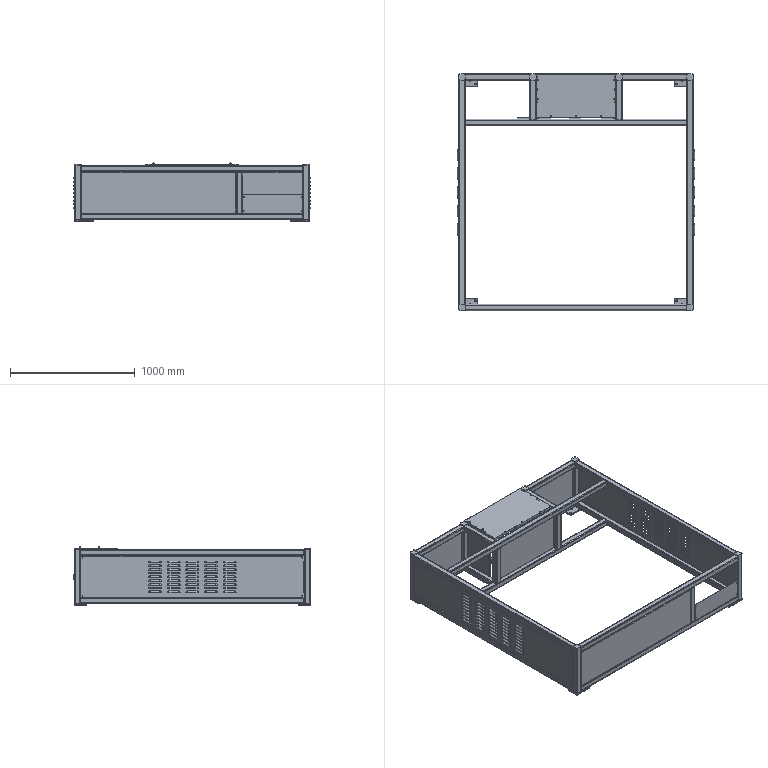Assembly | SolidWorks | mm | 51 component files | 55 solids | 2416 faces | box 1904 x 1905 x 472 mm | volume 47815882 mm3 | plane 1028 | cylinder 680 | sphere 392 | torus 188 | cone 128 | commonest cylinder face diameters 16 x120 6 x100 24 x90 4 x90 28 x90 8 x48 6.8 x32 4.5 x32
Bill of materials:
07.1.1 | 4 |  | Solid rectangular block, elongated, with all four long edges chamfered, giving an octagon-like end cross-section.
19.1.1 | 2 |  | Long, thin sheet-like panel with bent flanges on both long edges (C-shaped profile). It has a central field of raised louvers in five columns of about nine slots each, and small holes near the corners.
20.1.1 | 1 |  | Flat, thin rectangular plate with four oblong slots, two near each short end. It has no other visible features.
21.1.1 | 1 |  | Thin rectangular plate with slightly rounded edges and corners. A small, low raised pad or tab sits on one face, offset toward one edge.
22.1.1 | 1 |  | Thin rectangular plate with slightly rounded edges and corners. A small, low raised pad or tab sits on one face, offset toward one edge (the opposite end from the similar part).
23.1.1 | 1 |  | Plain thin rectangular plate with slightly rounded edges and corners. No holes or protrusions are visible.
24.1.1 | 2 |  | Rectangular sheet-like panel with partial-length folded flanges on all four edges, notched corners, and four small holes near the corners.
25.1.1 | 1 |  | Thin, flat rectangular strip with slightly rounded edges. No other features are visible.
09.1.1 | 4 |  | Long bar with a rectangular cross-section and chamfered longitudinal edges. One end is cut on an angle, tapering the bar's thickness at that end.
AX50x50-1_square tube.1.1 | 6 | AISI 1035 Steel (SS) | Straight prismatic bar with a square cross-section and large-radius rounded corners. It is moderately long compared to its width.
AX50x50-2_square tube.1.1 | 4 | AISI 1035 Steel (SS) | Long, slender, straight bar with a square cross-section and rounded corners. It has flat ends.
AX50x50-3_square tube.1.1 | 4 | AISI 1035 Steel (SS) | Long, slender, straight bar with a rounded-square cross-section and flat ends. Its shape looks very similar to unnamed part.
AX50x50-4_square tube.1.1 | 2 | AISI 1035 Steel (SS) | Long straight solid bar with a square cross-section and rounded longitudinal edges; flat square ends.
AX50x50-5_square tube.1.1 | 3 | AISI 1035 Steel (SS) | Straight solid bar with a square cross-section and rounded longitudinal edges, shown standing upright; flat ends.
AX50x50-6_square tube.1.1 | 4 | AISI 1035 Steel (SS) | Short straight solid bar with a square cross-section and rounded longitudinal edges; flat ends.
AX50x50-8_square tube.1.1 | 2 | AISI 1035 Steel (SS) | Long straight solid bar with a square cross-section and rounded longitudinal edges; flat square ends.
AXWHELL-PLATE.1.1 | 4 |  | Flat rectangular plate with rounded corners. It has four small round through-holes in a 2x2 rectangular pattern and one larger round through-hole near one corner.
04.1.1 | 1 |  | Large thin rectangular plate with slightly rounded corners. Four short tapered pins stick up from one face near the two short edges, and small through-holes run along the edges.
05.1.1 | 4 |  | Long thin flat rectangular strip with a constant thickness. One end is tapered at an angle in plan view, and the cross-section has small chamfered corners.
Mates:
1. coincident | assembly face at (1168.631, -386.636, 222.5) dir (0, 0, -1) | AX00-102.1.1-1/AX00-101.1.1-1/04.1.1-1 face at (-91.369, 1163.364, 222.5) dir (0, 0, 1)
2. coincident | assembly face at (-711.369, 1513.364, 222.5) dir (0, 1, 0) | AX00-102.1.1-1/AX00-101.1.1-1/04.1.1-1 face at (548.631, 1513.364, 222.5) dir (0, 1, 0)
3. coincident | assembly face at (1168.631, -386.636, 242.5) dir (0, 0, 1) | assembly face at (568.631, 1498.364, 242.5) dir (0, 0, -1)
4. coincident | assembly face at (-711.369, 1513.364, 222.5) dir (0, 1, 0) | assembly face at (568.631, 1513.364, 245.5) dir (0, 1, 0)
5. coincident | AX00-100.1.1-1/AXFrame_A.1.1-1/AX50x50-3_square tube.1.1-3 face at (1168.631, 1463.364, 212.5) dir (1, 0, 0) | assembly face at (1168.631, 1498.364, 242.5) dir (1, 0, 0)
6. coincident | AX00-100.1.1-1/AXFrame_A.1.1-1/AX50x50-2_square tube.1.1-5 face at (1118.631, 1148.364, 212.5) dir (0, 1, 0) | 07.1.1-2 face at (-241.369, 1148.364, 158.477) dir (0, -1, 0)
7. coincident | 07.1.1-1 face at (168.631, 1163.364, 188.477) dir (0, 1, 0) | 07.1.1-2 face at (-241.369, 1163.364, 158.477) dir (0, 1, 0)
8. coincident | 07.1.1-1 face at (268.631, 1163.364, 188.477) dir (0, 0, 1) | 07.1.1-2 face at (-141.369, 1148.364, 188.477) dir (0, 0, 1)
9. coincident | assembly face at (1168.631, -386.636, 242.5) dir (0, 0, 1) | assembly face at (261.596, 473.364, 242.5) dir (0, 0, -1)
10. coincident | assembly face at (531.631, 1473.364, 242.5) dir (0, -1, 0) | assembly face at (261.596, 473.364, 642.5) dir (0, 1, 0)
11. coincident | AXFrame_A.1.1-1/AX50x50-1_square tube.1.1-4 face at (1325.438, -406.343, 222.5) dir (1, 0, 0) | 19.1.1-1 face at (1325.438, -353.343, -171.5) dir (1, 0, 0)
12. distance | 19.1.1-1 face at (1323.438, -355.343, 119.5) dir (0, -1, 0) | AXFrame_A.1.1-1/AX50x50-1_square tube.1.1-4 face at (1275.438, -356.343, 222.5) dir (0, 1, 0)
13. distance | 19.1.1-1 face at (1323.438, 1398.657, 161.5) dir (0, 0, 1) | AXFrame_A.1.1-1/AX50x50-3_square tube.1.1-3 face at (1275.438, 1443.657, 162.5) dir (0, 0, -1)
14. coincident | AXFrame_A.1.1-1/AX50x50-1_square tube.1.1-3 face at (-554.562, -406.343, 222.5) dir (-1, 0, 0) | 19.1.1-2 face at (-554.562, 1440.657, -171.5) dir (-1, 0, 0)
15. distance | 19.1.1-2 face at (-552.562, -311.343, 161.5) dir (0, 0, 1) | AXFrame_A.1.1-1/AX50x50-3_square tube.1.1-1 face at (-554.562, 1443.657, 162.5) dir (0, 0, -1)
16. distance | 19.1.1-2 face at (-552.562, 1442.657, 119.5) dir (0, 1, 0) | AXFrame_A.1.1-1/AX50x50-1_square tube.1.1-6 face at (-554.562, 1443.657, 222.5) dir (0, -1, 0)
17. coincident | AXFrame_A.1.1-1/AX50x50-8_square tube.1.1-3 face at (755.438, 1493.657, -222.5) dir (0, 1, 0) | 21.1.1-1 face at (756.438, 1493.657, 161.5) dir (0, 1, 0)
18. distance | 21.1.1-1 face at (1274.438, 1493.657, 161.5) dir (0, 0, 1) | AXFrame_A.1.1-1/AX50x50-8_square tube.1.1-4 face at (755.438, 1443.657, 162.5) dir (0, 0, -1)
19. distance | 21.1.1-1 face at (756.438, 1493.657, -171.5) dir (-1, 0, 0) | AXFrame_A.1.1-1/AX50x50-1_square tube.1.1-7 face at (755.438, 1443.657, 222.5) dir (1, 0, 0)
20. coincident | AXFrame_A.1.1-1/AX50x50-4_square tube.1.1-3 face at (-504.562, 1493.657, -222.5) dir (0, 1, 0) | 22.1.1-2 face at (14.438, 1493.657, -171.5) dir (0, 1, 0)
21. distance | 22.1.1-2 face at (-503.562, 1493.657, 161.5) dir (-1, 0, 0) | AXFrame_A.1.1-1/AX50x50-1_square tube.1.1-6 face at (-504.562, 1443.657, 222.5) dir (1, 0, 0)
22. distance | 22.1.1-2 face at (-503.562, 1493.657, 161.5) dir (0, 0, 1) | AXFrame_A.1.1-1/AX50x50-4_square tube.1.1-4 face at (-504.562, 1443.657, 162.5) dir (0, 0, -1)
23. coincident | AXFrame_A.1.1-1/AX50x50-5_square tube.1.1-1 face at (15.438, 1128.657, 162.5) dir (0, 1, 0) | 23.1.1-1 face at (704.438, 1128.657, -170.5) dir (0, 1, 0)
24. coincident | AXFrame_A.1.1-1/AX50x50-2_square tube.1.1-5 face at (1275.438, 1078.657, 162.5) dir (0, 0, -1) | 23.1.1-1 face at (66.438, 1128.657, 162.5) dir (0, 0, 1)
25. distance | 23.1.1-1 face at (704.438, 1128.657, 162.5) dir (1, 0, 0) | AXFrame_A.1.1-1/AX50x50-5_square tube.1.1-2 face at (705.438, 1078.657, 162.5) dir (-1, 0, 0)
26. coincident | AXFrame_A.1.1-1/AX50x50-1_square tube.1.1-7 face at (705.438, 1443.657, 222.5) dir (-1, 0, 0) | 24.1.1-1 face at (705.438, 1374.657, -171.5) dir (-1, 0, 0)
27. distance | AXFrame_A.1.1-1/AX50x50-5_square tube.1.1-2 face at (705.438, 1128.657, 162.5) dir (0, 1, 0) | 24.1.1-1 face at (707.438, 1129.657, -129.5) dir (0, -1, 0)
28. distance | 24.1.1-1 face at (707.438, 1332.657, -171.5) dir (0, 0, -1) | AXFrame_A.1.1-1/AX50x50-6_square tube.1.1-4 face at (705.438, 1128.657, -172.5) dir (0, 0, 1)
29. coincident | AXFrame_A.1.1-1/AX50x50-1_square tube.1.1-8 face at (65.438, 1443.657, 222.5) dir (1, 0, 0) | 24.1.1-2 face at (65.438, 1197.657, -171.5) dir (1, 0, 0)
30. distance | 24.1.1-2 face at (63.438, 1398.657, 161.5) dir (0, 0, 1) | AXFrame_A.1.1-1/AX50x50-6_square tube.1.1-1 face at (15.438, 1128.657, 162.5) dir (0, 0, -1)
31. distance | 24.1.1-2 face at (63.438, 1442.657, -129.5) dir (0, 1, 0) | AXFrame_A.1.1-1/AX50x50-1_square tube.1.1-8 face at (15.438, 1443.657, 222.5) dir (0, -1, 0)
32. coincident | AXFrame_A.1.1-1/AX50x50-2_square tube.1.1-3 face at (1275.438, -406.343, -172.5) dir (0, -1, 0) | 25.1.1-1 face at (739.438, -406.343, 161.5) dir (0, -1, 0)
33. distance | 25.1.1-1 face at (-503.562, -406.343, -171.5) dir (-1, 0, 0) | AXFrame_A.1.1-1/AX50x50-1_square tube.1.1-3 face at (-504.562, -406.343, 222.5) dir (1, 0, 0)
34. distance | 25.1.1-1 face at (-503.562, -406.343, 161.5) dir (0, 0, 1) | AXFrame_A.1.1-1/AX50x50-2_square tube.1.1-2 face at (1275.438, -406.343, 162.5) dir (0, 0, -1)
35. coincident | AX50x50-1_square tube.1.1-3 face at (22.742, -23.319, 222.5) dir (1, 0, 0) | AX50x50-2_square tube.1.1-2 face at (22.742, 26.681, 162.5) dir (-1, 0, 0)
36. coincident | AX50x50-1_square tube.1.1-3 face at (-27.258, -23.319, 222.5) dir (0, -1, 0) | AX50x50-2_square tube.1.1-2 face at (1802.742, -23.319, 212.5) dir (0, -1, 0)
37. distance | AX50x50-1_square tube.1.1-3 face at (22.742, 26.681, 222.5) dir (0, 0, 1) | AX50x50-2_square tube.1.1-2 face at (1802.742, -23.319, 212.5) dir (0, 0, 1)
38. coincident | AX50x50-2_square tube.1.1-2 face at (1802.742, 26.681, 162.5) dir (1, 0, 0) | AX50x50-1_square tube.1.1-4 face at (1802.742, -23.319, 222.5) dir (-1, 0, 0)
39. coincident | AX50x50-2_square tube.1.1-2 face at (1802.742, -23.319, 212.5) dir (0, -1, 0) | AX50x50-1_square tube.1.1-4 face at (1802.742, -23.319, 222.5) dir (0, -1, 0)
40. coincident | AX50x50-1_square tube.1.1-3 face at (22.742, -23.319, 222.5) dir (1, 0, 0) | AX50x50-2_square tube.1.1-3 face at (22.742, 26.681, -222.5) dir (-1, 0, 0)
41. coincident | AX50x50-1_square tube.1.1-3 face at (-27.258, -23.319, 222.5) dir (0, -1, 0) | AX50x50-2_square tube.1.1-3 face at (1802.742, -23.319, -172.5) dir (0, -1, 0)
42. coincident | AX50x50-1_square tube.1.1-3 face at (22.742, 26.681, -222.5) dir (0, 0, -1) | AX50x50-2_square tube.1.1-3 face at (1802.742, -23.319, -222.5) dir (0, 0, -1)
43. coincident | AX50x50-1_square tube.1.1-3 face at (-27.258, 26.681, 222.5) dir (0, 1, 0) | AX50x50-3_square tube.1.1-1 face at (22.742, 26.681, 162.5) dir (0, -1, 0)
44. coincident | AX50x50-1_square tube.1.1-3 face at (-27.258, -23.319, 222.5) dir (-1, 0, 0) | AX50x50-3_square tube.1.1-1 face at (-27.258, 1826.681, 212.5) dir (-1, 0, 0)
45. distance | AX50x50-1_square tube.1.1-3 face at (22.742, 26.681, 222.5) dir (0, 0, 1) | AX50x50-3_square tube.1.1-1 face at (-27.258, 1826.681, 212.5) dir (0, 0, 1)
46. coincident | AX50x50-1_square tube.1.1-3 face at (-27.258, 26.681, 222.5) dir (0, 1, 0) | AX50x50-3_square tube.1.1-2 face at (22.742, 26.681, -222.5) dir (0, -1, 0)
47. coincident | AX50x50-1_square tube.1.1-3 face at (22.742, 26.681, -222.5) dir (0, 0, -1) | AX50x50-3_square tube.1.1-2 face at (-27.258, 1826.681, -222.5) dir (0, 0, -1)
48. coincident | AX50x50-1_square tube.1.1-3 face at (-27.258, -23.319, 222.5) dir (-1, 0, 0) | AX50x50-3_square tube.1.1-2 face at (-27.258, 1826.681, -172.5) dir (-1, 0, 0)
49. coincident | AX50x50-1_square tube.1.1-4 face at (1802.742, 26.681, 222.5) dir (0, 1, 0) | AX50x50-3_square tube.1.1-3 face at (1852.742, 26.681, 162.5) dir (0, -1, 0)
50. distance | AX50x50-1_square tube.1.1-4 face at (1852.742, 26.681, 222.5) dir (0, 0, 1) | AX50x50-3_square tube.1.1-3 face at (1802.742, 1826.681, 212.5) dir (0, 0, 1)
51. coincident | AX50x50-1_square tube.1.1-4 face at (1852.742, -23.319, 222.5) dir (1, 0, 0) | AX50x50-3_square tube.1.1-3 face at (1852.742, 1826.681, 212.5) dir (1, 0, 0)
52. coincident | AX50x50-1_square tube.1.1-4 face at (1852.742, -23.319, 222.5) dir (1, 0, 0) | AX50x50-3_square tube.1.1-4 face at (1852.742, 1826.681, -172.5) dir (1, 0, 0)
53. coincident | AX50x50-1_square tube.1.1-4 face at (1802.742, 26.681, 222.5) dir (0, 1, 0) | AX50x50-3_square tube.1.1-4 face at (1852.742, 26.681, -222.5) dir (0, -1, 0)
54. coincident | AX50x50-1_square tube.1.1-4 face at (1852.742, 26.681, -222.5) dir (0, 0, -1) | AX50x50-3_square tube.1.1-4 face at (1802.742, 1826.681, -222.5) dir (0, 0, -1)
55. coincident | AX50x50-1_square tube.1.1-3 face at (22.742, 26.681, -222.5) dir (0, 0, -1) | AX50x50-1_square tube.1.1-4 face at (1852.742, 26.681, -222.5) dir (0, 0, -1)
56. coincident | AX50x50-1_square tube.1.1-4 face at (1852.742, 26.681, 222.5) dir (0, 0, 1) | AX50x50-1_square tube.1.1-5 face at (1852.742, 1876.681, 222.5) dir (0, 0, 1)
57. coincident | AX50x50-3_square tube.1.1-3 face at (1852.742, 1826.681, 212.5) dir (1, 0, 0) | AX50x50-1_square tube.1.1-5 face at (1852.742, 1826.681, 222.5) dir (1, 0, 0)
58. coincident | AX50x50-3_square tube.1.1-3 face at (1852.742, 1826.681, 162.5) dir (0, 1, 0) | AX50x50-1_square tube.1.1-5 edge at (1810.742, 1826.681, 222.5) dir (0, 0, -1)
59. coincident | AX50x50-3_square tube.1.1-1 face at (22.742, 1826.681, 212.5) dir (1, 0, 0) | AX50x50-1_square tube.1.1-6 face at (22.742, 1826.681, 222.5) dir (1, 0, 0)
60. coincident | AX50x50-1_square tube.1.1-3 face at (22.742, 26.681, 222.5) dir (0, 0, 1) | AX50x50-1_square tube.1.1-6 face at (22.742, 1876.681, 222.5) dir (0, 0, 1)
61. coincident | AX50x50-3_square tube.1.1-1 face at (22.742, 1826.681, 162.5) dir (0, 1, 0) | AX50x50-1_square tube.1.1-6 face at (-27.258, 1826.681, 222.5) dir (0, -1, 0)
62. coincident | AX50x50-3_square tube.1.1-4 face at (1802.742, 1826.681, -172.5) dir (-1, 0, 0) | AX50x50-2_square tube.1.1-4 face at (1802.742, 1511.681, -222.5) dir (1, 0, 0)
63. coincident | AX50x50-3_square tube.1.1-4 face at (1802.742, 1826.681, -222.5) dir (0, 0, -1) | AX50x50-2_square tube.1.1-4 face at (1802.742, 1461.681, -222.5) dir (0, 0, -1)
64. coincident | AX50x50-3_square tube.1.1-3 face at (1802.742, 1826.681, 212.5) dir (-1, 0, 0) | AX50x50-2_square tube.1.1-5 face at (1802.742, 1511.681, 162.5) dir (1, 0, 0)
65. coincident | AX50x50-3_square tube.1.1-3 face at (1802.742, 1826.681, 212.5) dir (0, 0, 1) | AX50x50-2_square tube.1.1-5 face at (1802.742, 1461.681, 212.5) dir (0, 0, 1)
66. coincident | AX50x50-2_square tube.1.1-4 face at (1802.742, 1511.681, -172.5) dir (0, 1, 0) | AX50x50-2_square tube.1.1-5 face at (1802.742, 1511.681, 212.5) dir (0, 1, 0)
67. coincident | AX50x50-1_square tube.1.1-5 face at (1802.742, 1826.681, 222.5) dir (-1, 0, 0) | AX50x50-8_square tube.1.1-3 face at (1802.742, 1876.681, -172.5) dir (1, 0, 0)
68. coincident | AX50x50-1_square tube.1.1-5 face at (1802.742, 1876.681, 222.5) dir (0, 1, 0) | AX50x50-8_square tube.1.1-3 face at (1282.742, 1876.681, -222.5) dir (0, 1, 0)
69. coincident | AX50x50-1_square tube.1.1-5 face at (1852.742, 1876.681, -222.5) dir (0, 0, -1) | AX50x50-8_square tube.1.1-3 face at (1282.742, 1826.681, -222.5) dir (0, 0, -1)
70. coincident | AX50x50-1_square tube.1.1-5 face at (1802.742, 1876.681, 222.5) dir (0, 1, 0) | AX50x50-8_square tube.1.1-4 face at (1282.742, 1876.681, 162.5) dir (0, 1, 0)
71. coincident | AX50x50-1_square tube.1.1-5 face at (1802.742, 1826.681, 222.5) dir (-1, 0, 0) | AX50x50-8_square tube.1.1-4 face at (1802.742, 1876.681, 212.5) dir (1, 0, 0)
72. coincident | AX50x50-1_square tube.1.1-6 face at (-27.258, 1876.681, 222.5) dir (0, 1, 0) | AX50x50-4_square tube.1.1-3 face at (22.742, 1876.681, -222.5) dir (0, 1, 0)
73. coincident | AX50x50-1_square tube.1.1-6 face at (22.742, 1876.681, -222.5) dir (0, 0, -1) | AX50x50-4_square tube.1.1-3 face at (22.742, 1826.681, -222.5) dir (0, 0, -1)
74. coincident | AX50x50-1_square tube.1.1-6 face at (22.742, 1826.681, 222.5) dir (1, 0, 0) | AX50x50-4_square tube.1.1-3 face at (22.742, 1876.681, -172.5) dir (-1, 0, 0)
75. coincident | AX50x50-1_square tube.1.1-6 face at (22.742, 1826.681, 222.5) dir (1, 0, 0) | AX50x50-4_square tube.1.1-4 face at (22.742, 1876.681, 212.5) dir (-1, 0, 0)
76. coincident | AX50x50-1_square tube.1.1-6 face at (-27.258, 1876.681, 222.5) dir (0, 1, 0) | AX50x50-4_square tube.1.1-4 face at (22.742, 1876.681, 162.5) dir (0, 1, 0)
77. coincident | AX50x50-3_square tube.1.1-1 face at (-27.258, 1826.681, 212.5) dir (0, 0, 1) | AX50x50-4_square tube.1.1-4 face at (22.742, 1826.681, 212.5) dir (0, 0, 1)
78. coincident | AX50x50-3_square tube.1.1-3 face at (1802.742, 1826.681, 212.5) dir (0, 0, 1) | AX50x50-8_square tube.1.1-4 face at (1282.742, 1826.681, 212.5) dir (0, 0, 1)
79. coincident | AX50x50-1_square tube.1.1-5 face at (1852.742, 1876.681, 222.5) dir (0, 0, 1) | AX50x50-1_square tube.1.1-7 face at (1282.742, 1876.681, 222.5) dir (0, 0, 1)
80. coincident | AX50x50-8_square tube.1.1-4 face at (1282.742, 1876.681, 162.5) dir (0, 1, 0) | AX50x50-1_square tube.1.1-7 face at (1232.742, 1876.681, 222.5) dir (0, 1, 0)
81. coincident | AX50x50-8_square tube.1.1-4 face at (1282.742, 1876.681, 212.5) dir (-1, 0, 0) | AX50x50-1_square tube.1.1-7 face at (1282.742, 1826.681, 222.5) dir (1, 0, 0)
82. coincident | AX50x50-4_square tube.1.1-4 face at (22.742, 1876.681, 162.5) dir (0, 1, 0) | AX50x50-1_square tube.1.1-8 face at (542.742, 1876.681, 222.5) dir (0, 1, 0)
83. coincident | AX50x50-1_square tube.1.1-7 face at (1282.742, 1876.681, 222.5) dir (0, 0, 1) | AX50x50-1_square tube.1.1-8 face at (592.742, 1876.681, 222.5) dir (0, 0, 1)
84. coincident | AX50x50-4_square tube.1.1-4 face at (542.742, 1876.681, 212.5) dir (1, 0, 0) | AX50x50-1_square tube.1.1-8 face at (542.742, 1826.681, 222.5) dir (-1, 0, 0)
85. coincident | AX50x50-1_square tube.1.1-8 face at (542.742, 1826.681, 222.5) dir (0, -1, 0) | AX50x50-6_square tube.1.1-1 face at (592.742, 1826.681, 212.5) dir (0, 1, 0)
86. coincident | AX50x50-1_square tube.1.1-8 face at (592.742, 1826.681, 222.5) dir (1, 0, 0) | AX50x50-6_square tube.1.1-1 face at (592.742, 1511.681, 162.5) dir (1, 0, 0)
87. coincident | AX50x50-1_square tube.1.1-8 face at (542.742, 1826.681, 222.5) dir (0, -1, 0) | AX50x50-6_square tube.1.1-2 face at (592.742, 1826.681, -222.5) dir (0, 1, 0)
88. coincident | AX50x50-1_square tube.1.1-8 face at (592.742, 1826.681, 222.5) dir (1, 0, 0) | AX50x50-6_square tube.1.1-2 face at (592.742, 1511.681, -172.5) dir (1, 0, 0)
89. coincident | AX50x50-1_square tube.1.1-8 face at (592.742, 1876.681, -222.5) dir (0, 0, -1) | AX50x50-6_square tube.1.1-2 face at (542.742, 1511.681, -222.5) dir (0, 0, -1)
90. coincident | AX50x50-1_square tube.1.1-7 face at (1282.742, 1826.681, 222.5) dir (1, 0, 0) | AX50x50-6_square tube.1.1-3 face at (1282.742, 1511.681, 212.5) dir (1, 0, 0)
91. coincident | AX50x50-1_square tube.1.1-7 face at (1282.742, 1826.681, 222.5) dir (1, 0, 0) | AX50x50-6_square tube.1.1-4 face at (1282.742, 1511.681, -172.5) dir (1, 0, 0)
92. coincident | AX50x50-2_square tube.1.1-5 face at (1802.742, 1461.681, 212.5) dir (0, 0, 1) | AX50x50-6_square tube.1.1-1 face at (542.742, 1511.681, 212.5) dir (0, 0, 1)
93. coincident | AX50x50-1_square tube.1.1-7 face at (1232.742, 1826.681, 222.5) dir (0, -1, 0) | AX50x50-6_square tube.1.1-3 face at (1282.742, 1826.681, 162.5) dir (0, 1, 0)
94. coincident | AX50x50-2_square tube.1.1-5 face at (1802.742, 1461.681, 212.5) dir (0, 0, 1) | AX50x50-6_square tube.1.1-3 face at (1232.742, 1511.681, 212.5) dir (0, 0, 1)
95. coincident | AX50x50-1_square tube.1.1-7 face at (1232.742, 1826.681, 222.5) dir (0, -1, 0) | AX50x50-6_square tube.1.1-4 face at (1282.742, 1826.681, -222.5) dir (0, 1, 0)
96. coincident | AX50x50-1_square tube.1.1-7 face at (1282.742, 1876.681, -222.5) dir (0, 0, -1) | AX50x50-6_square tube.1.1-4 face at (1232.742, 1511.681, -222.5) dir (0, 0, -1)
97. coincident | AX50x50-2_square tube.1.1-4 face at (1802.742, 1511.681, -172.5) dir (0, 1, 0) | AX50x50-6_square tube.1.1-4 face at (1282.742, 1511.681, -222.5) dir (0, -1, 0)
98. coincident | AX50x50-2_square tube.1.1-4 face at (1802.742, 1511.681, -172.5) dir (0, 1, 0) | AX50x50-5_square tube.1.1-1 face at (542.742, 1511.681, 162.5) dir (0, 1, 0)
99. coincident | AX50x50-6_square tube.1.1-2 face at (592.742, 1511.681, -172.5) dir (1, 0, 0) | AX50x50-5_square tube.1.1-1 face at (592.742, 1461.681, 162.5) dir (1, 0, 0)
100. coincident | AX50x50-2_square tube.1.1-4 face at (1802.742, 1461.681, -172.5) dir (0, 0, 1) | AX50x50-5_square tube.1.1-1 face at (592.742, 1511.681, -172.5) dir (0, 0, -1)
101. coincident | AX50x50-2_square tube.1.1-4 face at (1802.742, 1511.681, -172.5) dir (0, 1, 0) | AX50x50-5_square tube.1.1-2 face at (1232.742, 1511.681, 162.5) dir (0, 1, 0)
102. coincident | AX50x50-2_square tube.1.1-4 face at (1802.742, 1461.681, -172.5) dir (0, 0, 1) | AX50x50-5_square tube.1.1-2 face at (1282.742, 1511.681, -172.5) dir (0, 0, -1)
103. coincident | AX50x50-6_square tube.1.1-3 face at (1232.742, 1511.681, 212.5) dir (-1, 0, 0) | AX50x50-5_square tube.1.1-2 face at (1232.742, 1461.681, 162.5) dir (-1, 0, 0)
104. coincident | AX50x50-1_square tube.1.1-4 face at (1852.742, 26.681, -222.5) dir (0, 0, -1) | AXwheel-assembly-2.1.1-2/AXWHELL-PLATE.1.1-1 face at (1852.742, -23.319, -222.5) dir (0, 0, 1)
105. coincident | AX50x50-1_square tube.1.1-4 face at (1802.742, -23.319, 222.5) dir (0, -1, 0) | AXwheel-assembly-2.1.1-2/AXWHELL-PLATE.1.1-1 face at (1702.742, -23.319, -222.5) dir (0, -1, 0)
106. coincident | AX50x50-1_square tube.1.1-4 face at (1852.742, -23.319, 222.5) dir (1, 0, 0) | AXwheel-assembly-2.1.1-2/AXWHELL-PLATE.1.1-1 face at (1852.742, -23.319, -222.5) dir (1, 0, 0)
107. coincident | AX50x50-1_square tube.1.1-3 face at (22.742, 26.681, -222.5) dir (0, 0, -1) | AXwheel-assembly-1.1.1-2/AXWHELL-PLATE.1.1-1 face at (-27.258, -23.319, -222.5) dir (0, 0, 1)
108. coincident | AX50x50-1_square tube.1.1-3 face at (-27.258, -23.319, 222.5) dir (0, -1, 0) | AXwheel-assembly-1.1.1-2/AXWHELL-PLATE.1.1-1 face at (122.742, -23.319, -234.5) dir (0, -1, 0)
109. coincident | AX50x50-1_square tube.1.1-3 face at (-27.258, -23.319, 222.5) dir (-1, 0, 0) | AXwheel-assembly-1.1.1-2/AXWHELL-PLATE.1.1-1 face at (-27.258, -23.319, -234.5) dir (-1, 0, 0)
110. coincident | AX50x50-1_square tube.1.1-6 face at (22.742, 1876.681, -222.5) dir (0, 0, -1) | AXwheel-assembly-3.1.1-2/AXWHELL-PLATE.1.1-1 face at (-27.258, 1876.681, -222.5) dir (0, 0, 1)
111. coincident | AX50x50-1_square tube.1.1-6 face at (-27.258, 1826.681, 222.5) dir (-1, 0, 0) | AXwheel-assembly-3.1.1-2/AXWHELL-PLATE.1.1-1 face at (-27.258, 1876.681, -222.5) dir (-1, 0, 0)
112. coincident | AX50x50-1_square tube.1.1-6 face at (-27.258, 1876.681, 222.5) dir (0, 1, 0) | AXwheel-assembly-3.1.1-2/AXWHELL-PLATE.1.1-1 face at (122.742, 1876.681, -222.5) dir (0, 1, 0)
113. coincident | AX50x50-1_square tube.1.1-5 face at (1852.742, 1876.681, -222.5) dir (0, 0, -1) | AXwheel-assembly-4.1.1-2/AXWHELL-PLATE.1.1-1 face at (1852.742, 1876.681, -222.5) dir (0, 0, 1)
114. coincident | AX50x50-1_square tube.1.1-5 face at (1852.742, 1826.681, 222.5) dir (1, 0, 0) | AXwheel-assembly-4.1.1-2/AXWHELL-PLATE.1.1-1 face at (1852.742, 1876.681, -234.5) dir (1, 0, 0)
115. coincident | AX50x50-1_square tube.1.1-5 face at (1802.742, 1876.681, 222.5) dir (0, 1, 0) | AXwheel-assembly-4.1.1-2/AXWHELL-PLATE.1.1-1 face at (1702.742, 1876.681, -234.5) dir (0, 1, 0)
116. coincident | AX50x50-2_square tube.1.1-2 face at (1802.742, -23.319, 162.5) dir (0, 0, -1) | AX50x50-5_square tube.1.1-3 face at (1317.742, -23.319, 162.5) dir (0, 0, 1)
117. coincident | AX50x50-2_square tube.1.1-3 face at (1802.742, -23.319, -172.5) dir (0, -1, 0) | AX50x50-5_square tube.1.1-3 face at (1267.742, -23.319, 162.5) dir (0, -1, 0)
118. distance | AX50x50-1_square tube.1.1-4 face at (1802.742, -23.319, 222.5) dir (-1, 0, 0) | AX50x50-5_square tube.1.1-3 face at (1317.742, 26.681, 162.5) dir (1, 0, 0)
119. coincident | AX50x50-1_square tube.1.1-8 face at (592.742, 1826.681, 222.5) dir (1, 0, 0) | 09.1.1-1 face at (592.742, 1876.681, 182.5) dir (-1, 0, 0)
120. distance | 09.1.1-1 face at (607.742, 1511.681, 182.5) dir (0, 0, 1) | AX50x50-6_square tube.1.1-1 face at (542.742, 1511.681, 212.5) dir (0, 0, 1)
121. coincident | AX50x50-1_square tube.1.1-8 face at (542.742, 1876.681, 222.5) dir (0, 1, 0) | 09.1.1-1 face at (607.742, 1876.681, 152.5) dir (0, 1, 0)
122. coincident | AX50x50-1_square tube.1.1-8 face at (592.742, 1826.681, 222.5) dir (1, 0, 0) | 09.1.1-2 face at (592.742, 1876.681, -17.5) dir (-1, 0, 0)
123. distance | 09.1.1-2 face at (607.742, 1511.681, -17.5) dir (0, 0, 1) | 09.1.1-1 face at (607.742, 1511.681, 182.5) dir (0, 0, 1)
124. coincident | AX50x50-1_square tube.1.1-8 face at (542.742, 1876.681, 222.5) dir (0, 1, 0) | 09.1.1-2 face at (607.742, 1876.681, -47.5) dir (0, 1, 0)
125. coincident | AX50x50-1_square tube.1.1-7 face at (1232.742, 1826.681, 222.5) dir (-1, 0, 0) | 09.1.1-3 face at (1232.742, 1876.681, 152.5) dir (1, 0, 0)
126. coincident | 09.1.1-1 face at (607.742, 1511.681, 182.5) dir (0, 0, 1) | 09.1.1-3 face at (1217.742, 1511.681, 182.5) dir (0, 0, 1)
127. coincident | AX50x50-1_square tube.1.1-7 face at (1232.742, 1876.681, 222.5) dir (0, 1, 0) | 09.1.1-3 face at (1217.742, 1876.681, 182.5) dir (0, 1, 0)
128. coincident | AX50x50-1_square tube.1.1-7 face at (1232.742, 1826.681, 222.5) dir (-1, 0, 0) | 09.1.1-4 face at (1232.742, 1876.681, -47.5) dir (1, 0, 0)
129. coincident | AX50x50-1_square tube.1.1-7 face at (1232.742, 1876.681, 222.5) dir (0, 1, 0) | 09.1.1-4 face at (1217.742, 1876.681, -17.5) dir (0, 1, 0)
130. coincident | 09.1.1-2 face at (607.742, 1511.681, -17.5) dir (0, 0, 1) | 09.1.1-4 face at (1217.742, 1511.681, -17.5) dir (0, 0, 1)
131. distance | 05.1.1-1 face at (290.831, -142.809, 192.5) dir (0, 0, 1) | 04.1.1-1 face at (305.831, 207.191, 232.5) dir (0, 0, 1)
132. distance | 05.1.1-2 face at (290.831, -142.809, -7.5) dir (0, 0, 1) | 05.1.1-1 face at (290.831, -142.809, 192.5) dir (0, 0, 1)
133. coincident | 05.1.1-3 face at (-304.169, 197.191, 162.5) dir (1, 0, 0) | 05.1.1-4 face at (-304.169, 197.191, -37.5) dir (1, 0, 0)
134. coincident | 05.1.1-3 face at (-319.169, -142.809, 192.5) dir (0, -1, 0) | 05.1.1-4 face at (-319.169, -142.809, -7.5) dir (0, -1, 0)
135. coincident | 05.1.1-1 face at (290.831, -142.809, 192.5) dir (0, 0, 1) | 05.1.1-3 face at (-319.169, -142.809, 192.5) dir (0, 0, 1)
136. coincident | 05.1.1-2 face at (290.831, -142.809, -7.5) dir (0, 0, 1) | 05.1.1-4 face at (-319.169, -142.809, -7.5) dir (0, 0, 1)
137. coincident | 05.1.1-3 face at (-319.169, -142.809, 192.5) dir (0, 0, 1) | 07.1.1-1 face at (-314.169, 207.191, 192.5) dir (0, 0, 1)
138. coincident | 05.1.1-1 face at (290.831, -142.809, 192.5) dir (0, 0, 1) | 07.1.1-2 face at (185.831, 207.191, 192.5) dir (0, 0, 1)